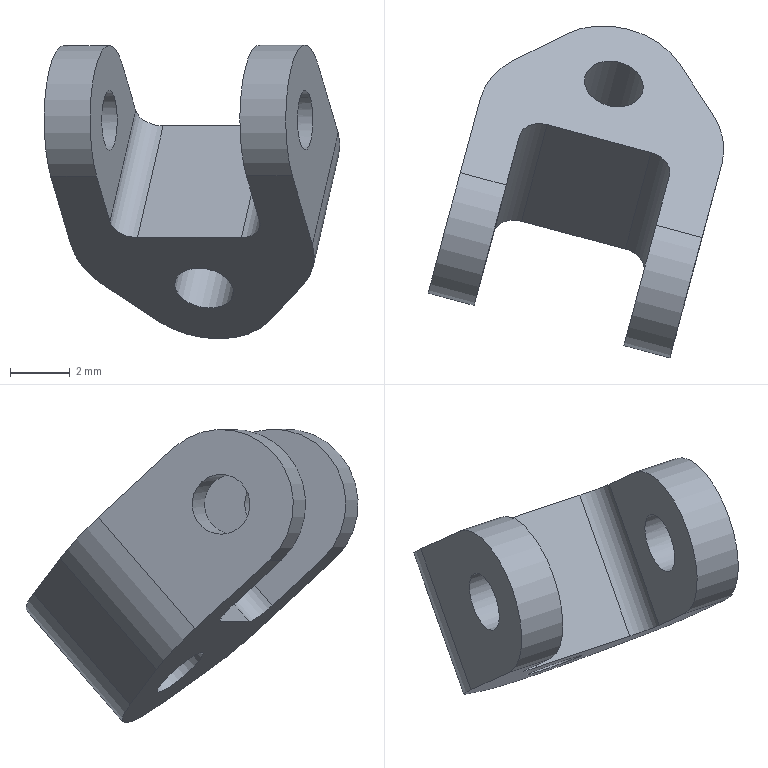Component | NX | UNIVERSAL_JOINT_1 | 1 solid | 19 faces | volume 211 mm3 | cylinder 10 | plane 9 | commonest cylinder face diameters 2 x3 6.35 x2 1.587 x2 5 x2 5.08 x1